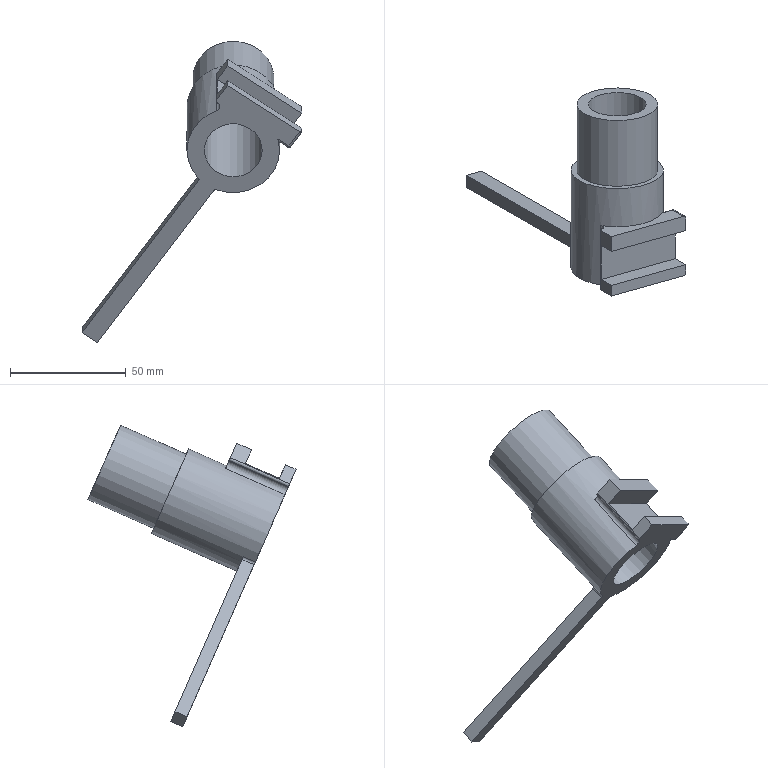Component | NX | ZHOU_PEI | 1 solid | 31 faces | volume 56172 mm3 | plane 17 | cylinder 12 | sphere 2 | commonest cylinder face diameters 2 x8 40 x1 35 x1 25 x1 4 x1